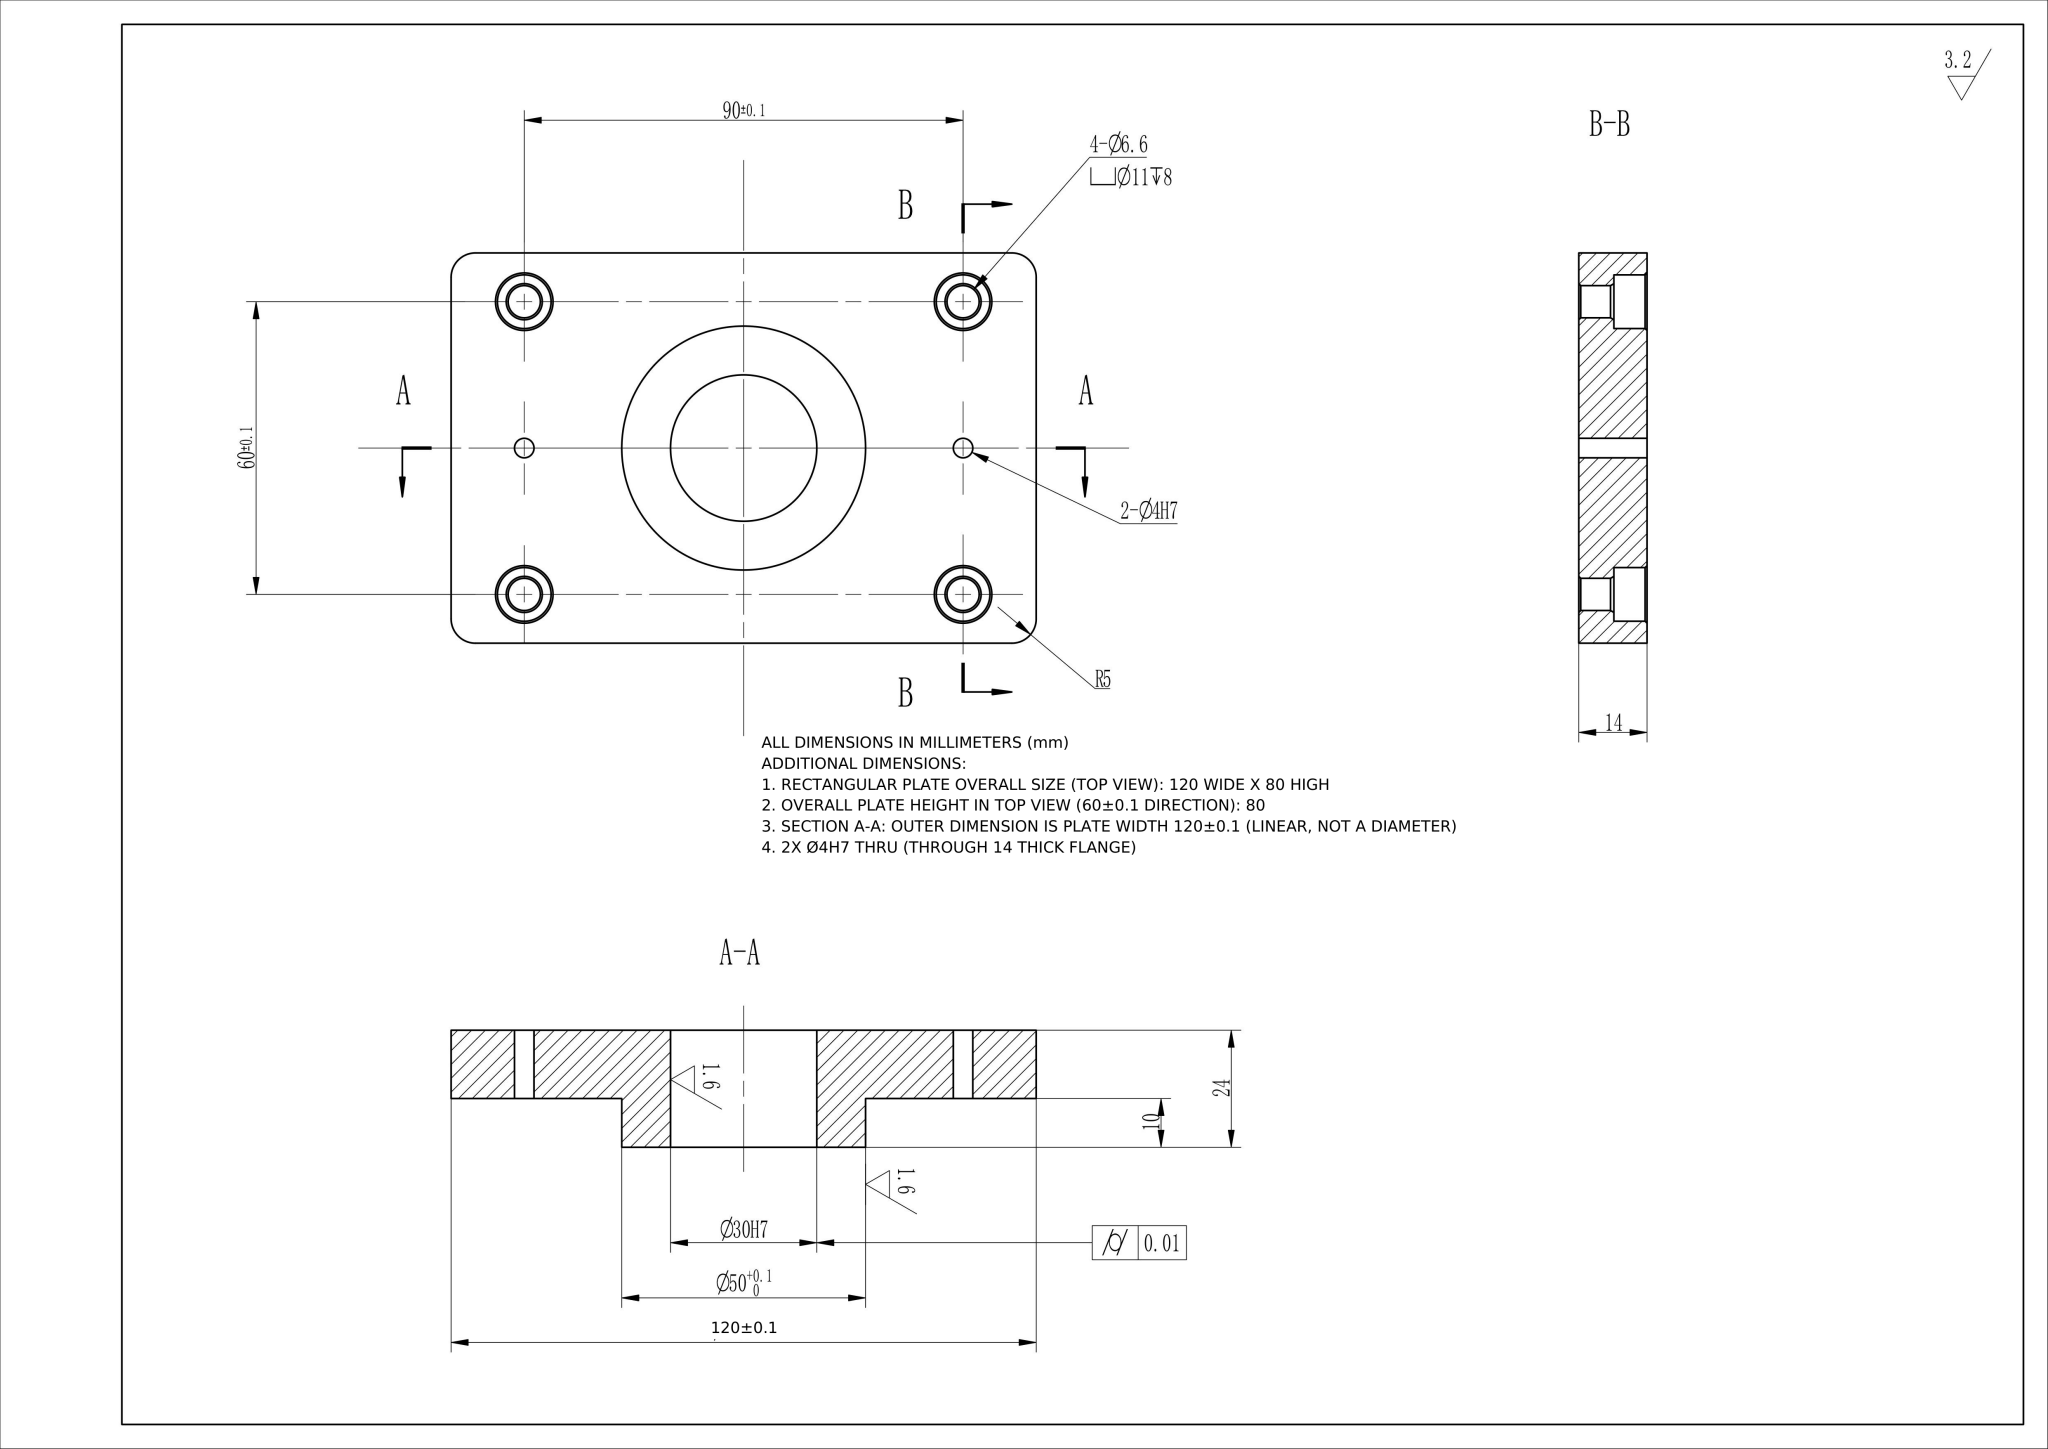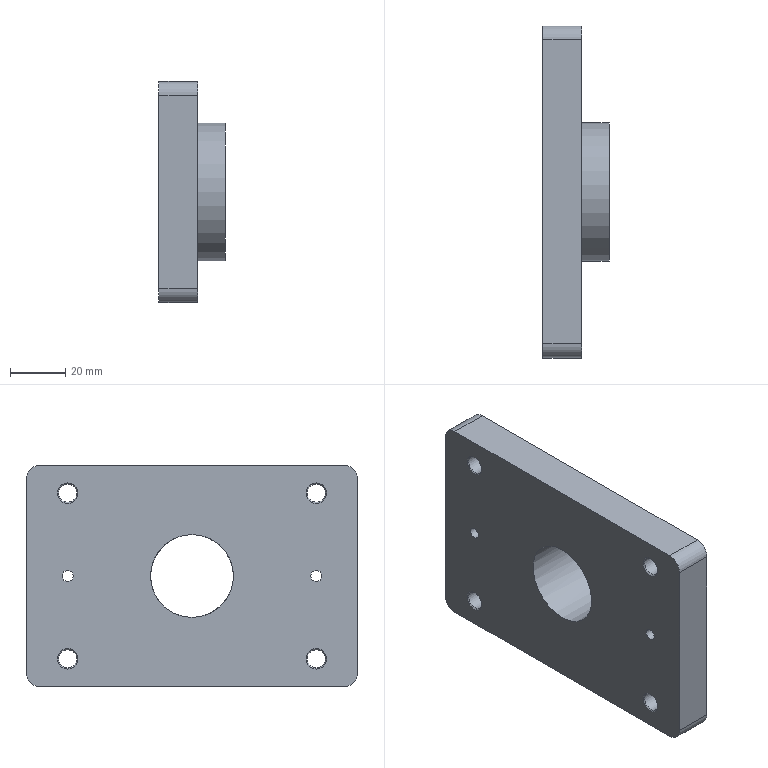Part | NX | mm | 1 solid | 39 faces | box 24 x 120 x 80 mm | volume 132818 mm3 | cylinder 16 | cone 12 | plane 11 | commonest cylinder face diameters 6.6 x4 11 x4 10 x4 4 x2 50 x1 30 x1
STEP:
#1=CARTESIAN_POINT('',(0.,0.,0.));
#2=DIRECTION('',(0.,0.,1.));
#3=DIRECTION('',(1.,0.,0.));
#4=AXIS2_PLACEMENT_3D('',#1,#2,#3);
#5=(LENGTH_UNIT()NAMED_UNIT(*)SI_UNIT(.MILLI.,.METRE.));
#6=UNCERTAINTY_MEASURE_WITH_UNIT(LENGTH_MEASURE(0.00002),#5,'','');
#7=(NAMED_UNIT(*)PLANE_ANGLE_UNIT()SI_UNIT($,.RADIAN.));
#8=PLANE_ANGLE_MEASURE_WITH_UNIT(PLANE_ANGLE_MEASURE(0.01745),#7);
#9=DIMENSIONAL_EXPONENTS(0.,0.,0.,0.,0.,0.,0.);
#10=(CONVERSION_BASED_UNIT('',#8)NAMED_UNIT(#9)PLANE_ANGLE_UNIT());
#11=(NAMED_UNIT(*)SI_UNIT($,.STERADIAN.)SOLID_ANGLE_UNIT());
#12=(GEOMETRIC_REPRESENTATION_CONTEXT(3)GLOBAL_UNCERTAINTY_ASSIGNED_CONTEXT((#6))GLOBAL_UNIT_ASSIGNED_CONTEXT((#5,#10,#11))REPRESENTATION_CONTEXT('',''));
#13=SHAPE_REPRESENTATION('',(#4),#12);
#14=CARTESIAN_POINT('',(0.,-60.,35.));
#15=VERTEX_POINT('',#14);
#16=CARTESIAN_POINT('',(0.,-60.,-35.));
#17=VERTEX_POINT('',#16);
#18=CARTESIAN_POINT('',(0.,-60.,40.));
#19=DIRECTION('',(0.,0.,-1.));
#20=VECTOR('',#19,1.);
#21=LINE('',#18,#20);
#22=EDGE_CURVE('',#15,#17,#21,.T.);
#23=ORIENTED_EDGE('',*,*,#22,.T.);
#24=CARTESIAN_POINT('',(14.,-60.,-35.));
#25=VERTEX_POINT('',#24);
#26=CARTESIAN_POINT('',(14.,-60.,-35.));
#27=DIRECTION('',(1.,0.,0.));
#28=VECTOR('',#27,1.);
#29=LINE('',#26,#28);
#30=EDGE_CURVE('',#17,#25,#29,.T.);
#31=ORIENTED_EDGE('',*,*,#30,.T.);
#32=CARTESIAN_POINT('',(14.,-60.,35.));
#33=VERTEX_POINT('',#32);
#34=CARTESIAN_POINT('',(14.,-60.,40.));
#35=DIRECTION('',(0.,0.,-1.));
#36=VECTOR('',#35,1.);
#37=LINE('',#34,#36);
#38=EDGE_CURVE('',#33,#25,#37,.T.);
#39=ORIENTED_EDGE('',*,*,#38,.F.);
#40=CARTESIAN_POINT('',(14.,-60.,35.));
#41=DIRECTION('',(-1.,0.,0.));
#42=VECTOR('',#41,1.);
#43=LINE('',#40,#42);
#44=EDGE_CURVE('',#33,#15,#43,.T.);
#45=ORIENTED_EDGE('',*,*,#44,.T.);
#46=EDGE_LOOP('',(#23,#31,#39,#45));
#47=FACE_OUTER_BOUND('',#46,.T.);
#48=CARTESIAN_POINT('',(14.,-60.,40.));
#49=DIRECTION('',(0.,1.,0.));
#50=DIRECTION('',(0.,0.,1.));
#51=AXIS2_PLACEMENT_3D('',#48,#49,#50);
#52=PLANE('',#51);
#53=ADVANCED_FACE('',(#47),#52,.F.);
#54=CARTESIAN_POINT('',(0.,-55.,-40.));
#55=VERTEX_POINT('',#54);
#56=CARTESIAN_POINT('',(0.,55.,-40.));
#57=VERTEX_POINT('',#56);
#58=CARTESIAN_POINT('',(0.,-60.,-40.));
#59=DIRECTION('',(0.,1.,0.));
#60=VECTOR('',#59,1.);
#61=LINE('',#58,#60);
#62=EDGE_CURVE('',#55,#57,#61,.T.);
#63=ORIENTED_EDGE('',*,*,#62,.T.);
#64=CARTESIAN_POINT('',(14.,55.,-40.));
#65=VERTEX_POINT('',#64);
#66=CARTESIAN_POINT('',(14.,55.,-40.));
#67=DIRECTION('',(1.,0.,0.));
#68=VECTOR('',#67,1.);
#69=LINE('',#66,#68);
#70=EDGE_CURVE('',#57,#65,#69,.T.);
#71=ORIENTED_EDGE('',*,*,#70,.T.);
#72=CARTESIAN_POINT('',(14.,-55.,-40.));
#73=VERTEX_POINT('',#72);
#74=CARTESIAN_POINT('',(14.,-60.,-40.));
#75=DIRECTION('',(0.,1.,0.));
#76=VECTOR('',#75,1.);
#77=LINE('',#74,#76);
#78=EDGE_CURVE('',#73,#65,#77,.T.);
#79=ORIENTED_EDGE('',*,*,#78,.F.);
#80=CARTESIAN_POINT('',(14.,-55.,-40.));
#81=DIRECTION('',(-1.,0.,0.));
#82=VECTOR('',#81,1.);
#83=LINE('',#80,#82);
#84=EDGE_CURVE('',#73,#55,#83,.T.);
#85=ORIENTED_EDGE('',*,*,#84,.T.);
#86=EDGE_LOOP('',(#63,#71,#79,#85));
#87=FACE_OUTER_BOUND('',#86,.T.);
#88=CARTESIAN_POINT('',(14.,-60.,-40.));
#89=DIRECTION('',(0.,0.,1.));
#90=DIRECTION('',(1.,0.,0.));
#91=AXIS2_PLACEMENT_3D('',#88,#89,#90);
#92=PLANE('',#91);
#93=ADVANCED_FACE('',(#87),#92,.F.);
#94=CARTESIAN_POINT('',(14.,60.,-35.));
#95=VERTEX_POINT('',#94);
#96=CARTESIAN_POINT('',(14.,60.,35.));
#97=VERTEX_POINT('',#96);
#98=CARTESIAN_POINT('',(14.,60.,-40.));
#99=DIRECTION('',(0.,0.,1.));
#100=VECTOR('',#99,1.);
#101=LINE('',#98,#100);
#102=EDGE_CURVE('',#95,#97,#101,.T.);
#103=ORIENTED_EDGE('',*,*,#102,.F.);
#104=CARTESIAN_POINT('',(0.,60.,-35.));
#105=VERTEX_POINT('',#104);
#106=CARTESIAN_POINT('',(14.,60.,-35.));
#107=DIRECTION('',(-1.,0.,0.));
#108=VECTOR('',#107,1.);
#109=LINE('',#106,#108);
#110=EDGE_CURVE('',#95,#105,#109,.T.);
#111=ORIENTED_EDGE('',*,*,#110,.T.);
#112=CARTESIAN_POINT('',(0.,60.,35.));
#113=VERTEX_POINT('',#112);
#114=CARTESIAN_POINT('',(0.,60.,-40.));
#115=DIRECTION('',(0.,0.,1.));
#116=VECTOR('',#115,1.);
#117=LINE('',#114,#116);
#118=EDGE_CURVE('',#105,#113,#117,.T.);
#119=ORIENTED_EDGE('',*,*,#118,.T.);
#120=CARTESIAN_POINT('',(14.,60.,35.));
#121=DIRECTION('',(1.,0.,0.));
#122=VECTOR('',#121,1.);
#123=LINE('',#120,#122);
#124=EDGE_CURVE('',#113,#97,#123,.T.);
#125=ORIENTED_EDGE('',*,*,#124,.T.);
#126=EDGE_LOOP('',(#103,#111,#119,#125));
#127=FACE_OUTER_BOUND('',#126,.T.);
#128=CARTESIAN_POINT('',(14.,60.,-40.));
#129=DIRECTION('',(0.,-1.,0.));
#130=DIRECTION('',(0.,0.,-1.));
#131=AXIS2_PLACEMENT_3D('',#128,#129,#130);
#132=PLANE('',#131);
#133=ADVANCED_FACE('',(#127),#132,.F.);
#134=CARTESIAN_POINT('',(14.,55.,40.));
#135=VERTEX_POINT('',#134);
#136=CARTESIAN_POINT('',(14.,-55.,40.));
#137=VERTEX_POINT('',#136);
#138=CARTESIAN_POINT('',(14.,60.,40.));
#139=DIRECTION('',(0.,-1.,0.));
#140=VECTOR('',#139,1.);
#141=LINE('',#138,#140);
#142=EDGE_CURVE('',#135,#137,#141,.T.);
#143=ORIENTED_EDGE('',*,*,#142,.F.);
#144=CARTESIAN_POINT('',(0.,55.,40.));
#145=VERTEX_POINT('',#144);
#146=CARTESIAN_POINT('',(14.,55.,40.));
#147=DIRECTION('',(-1.,0.,0.));
#148=VECTOR('',#147,1.);
#149=LINE('',#146,#148);
#150=EDGE_CURVE('',#135,#145,#149,.T.);
#151=ORIENTED_EDGE('',*,*,#150,.T.);
#152=CARTESIAN_POINT('',(0.,-55.,40.));
#153=VERTEX_POINT('',#152);
#154=CARTESIAN_POINT('',(0.,60.,40.));
#155=DIRECTION('',(0.,-1.,0.));
#156=VECTOR('',#155,1.);
#157=LINE('',#154,#156);
#158=EDGE_CURVE('',#145,#153,#157,.T.);
#159=ORIENTED_EDGE('',*,*,#158,.T.);
#160=CARTESIAN_POINT('',(14.,-55.,40.));
#161=DIRECTION('',(1.,0.,0.));
#162=VECTOR('',#161,1.);
#163=LINE('',#160,#162);
#164=EDGE_CURVE('',#153,#137,#163,.T.);
#165=ORIENTED_EDGE('',*,*,#164,.T.);
#166=EDGE_LOOP('',(#143,#151,#159,#165));
#167=FACE_OUTER_BOUND('',#166,.T.);
#168=CARTESIAN_POINT('',(14.,60.,40.));
#169=DIRECTION('',(0.,0.,-1.));
#170=DIRECTION('',(-1.,0.,0.));
#171=AXIS2_PLACEMENT_3D('',#168,#169,#170);
#172=PLANE('',#171);
#173=ADVANCED_FACE('',(#167),#172,.F.);
#174=CARTESIAN_POINT('',(14.,45.,2.));
#175=VERTEX_POINT('',#174);
#176=CARTESIAN_POINT('',(14.,45.,0.));
#177=DIRECTION('',(-1.,0.,0.));
#178=DIRECTION('',(0.,0.,1.));
#179=AXIS2_PLACEMENT_3D('',#176,#177,#178);
#180=CIRCLE('',#179,2.);
#181=EDGE_CURVE('',#175,#175,#180,.T.);
#182=ORIENTED_EDGE('',*,*,#181,.T.);
#183=EDGE_LOOP('',(#182));
#184=FACE_BOUND('',#183,.T.);
#185=CARTESIAN_POINT('',(14.,-45.,2.));
#186=VERTEX_POINT('',#185);
#187=CARTESIAN_POINT('',(14.,-45.,0.));
#188=DIRECTION('',(-1.,0.,0.));
#189=DIRECTION('',(0.,0.,1.));
#190=AXIS2_PLACEMENT_3D('',#187,#188,#189);
#191=CIRCLE('',#190,2.);
#192=EDGE_CURVE('',#186,#186,#191,.T.);
#193=ORIENTED_EDGE('',*,*,#192,.T.);
#194=EDGE_LOOP('',(#193));
#195=FACE_BOUND('',#194,.T.);
#196=CARTESIAN_POINT('',(14.,25.,-0.));
#197=VERTEX_POINT('',#196);
#198=CARTESIAN_POINT('',(14.,0.,0.));
#199=DIRECTION('',(1.,0.,0.));
#200=DIRECTION('',(0.,1.,-0.));
#201=AXIS2_PLACEMENT_3D('',#198,#199,#200);
#202=CIRCLE('',#201,25.);
#203=EDGE_CURVE('',#197,#197,#202,.T.);
#204=ORIENTED_EDGE('',*,*,#203,.F.);
#205=EDGE_LOOP('',(#204));
#206=FACE_BOUND('',#205,.T.);
#207=CARTESIAN_POINT('',(14.,45.,-35.9));
#208=VERTEX_POINT('',#207);
#209=CARTESIAN_POINT('',(14.,45.,-30.));
#210=DIRECTION('',(-1.,0.,0.));
#211=DIRECTION('',(0.,0.,-1.));
#212=AXIS2_PLACEMENT_3D('',#209,#210,#211);
#213=CIRCLE('',#212,5.9);
#214=EDGE_CURVE('',#208,#208,#213,.T.);
#215=ORIENTED_EDGE('',*,*,#214,.T.);
#216=EDGE_LOOP('',(#215));
#217=FACE_BOUND('',#216,.T.);
#218=CARTESIAN_POINT('',(14.,-45.,-35.9));
#219=VERTEX_POINT('',#218);
#220=CARTESIAN_POINT('',(14.,-45.,-30.));
#221=DIRECTION('',(-1.,0.,0.));
#222=DIRECTION('',(0.,0.,-1.));
#223=AXIS2_PLACEMENT_3D('',#220,#221,#222);
#224=CIRCLE('',#223,5.9);
#225=EDGE_CURVE('',#219,#219,#224,.T.);
#226=ORIENTED_EDGE('',*,*,#225,.T.);
#227=EDGE_LOOP('',(#226));
#228=FACE_BOUND('',#227,.T.);
#229=CARTESIAN_POINT('',(14.,45.,24.1));
#230=VERTEX_POINT('',#229);
#231=CARTESIAN_POINT('',(14.,45.,30.));
#232=DIRECTION('',(-1.,0.,0.));
#233=DIRECTION('',(0.,0.,-1.));
#234=AXIS2_PLACEMENT_3D('',#231,#232,#233);
#235=CIRCLE('',#234,5.9);
#236=EDGE_CURVE('',#230,#230,#235,.T.);
#237=ORIENTED_EDGE('',*,*,#236,.T.);
#238=EDGE_LOOP('',(#237));
#239=FACE_BOUND('',#238,.T.);
#240=CARTESIAN_POINT('',(14.,-45.,24.1));
#241=VERTEX_POINT('',#240);
#242=CARTESIAN_POINT('',(14.,-45.,30.));
#243=DIRECTION('',(-1.,0.,0.));
#244=DIRECTION('',(0.,0.,-1.));
#245=AXIS2_PLACEMENT_3D('',#242,#243,#244);
#246=CIRCLE('',#245,5.9);
#247=EDGE_CURVE('',#241,#241,#246,.T.);
#248=ORIENTED_EDGE('',*,*,#247,.T.);
#249=EDGE_LOOP('',(#248));
#250=FACE_BOUND('',#249,.T.);
#251=ORIENTED_EDGE('',*,*,#78,.T.);
#252=CARTESIAN_POINT('',(14.,55.,-35.));
#253=DIRECTION('',(1.,0.,0.));
#254=DIRECTION('',(0.,0.,-1.));
#255=AXIS2_PLACEMENT_3D('',#252,#253,#254);
#256=CIRCLE('',#255,5.);
#257=EDGE_CURVE('',#65,#95,#256,.T.);
#258=ORIENTED_EDGE('',*,*,#257,.T.);
#259=ORIENTED_EDGE('',*,*,#102,.T.);
#260=CARTESIAN_POINT('',(14.,55.,35.));
#261=DIRECTION('',(1.,0.,0.));
#262=DIRECTION('',(0.,0.,-1.));
#263=AXIS2_PLACEMENT_3D('',#260,#261,#262);
#264=CIRCLE('',#263,5.);
#265=EDGE_CURVE('',#97,#135,#264,.T.);
#266=ORIENTED_EDGE('',*,*,#265,.T.);
#267=ORIENTED_EDGE('',*,*,#142,.T.);
#268=CARTESIAN_POINT('',(14.,-55.,35.));
#269=DIRECTION('',(1.,0.,0.));
#270=DIRECTION('',(0.,0.,-1.));
#271=AXIS2_PLACEMENT_3D('',#268,#269,#270);
#272=CIRCLE('',#271,5.);
#273=EDGE_CURVE('',#137,#33,#272,.T.);
#274=ORIENTED_EDGE('',*,*,#273,.T.);
#275=ORIENTED_EDGE('',*,*,#38,.T.);
#276=CARTESIAN_POINT('',(14.,-55.,-35.));
#277=DIRECTION('',(1.,0.,0.));
#278=DIRECTION('',(0.,0.,-1.));
#279=AXIS2_PLACEMENT_3D('',#276,#277,#278);
#280=CIRCLE('',#279,5.);
#281=EDGE_CURVE('',#25,#73,#280,.T.);
#282=ORIENTED_EDGE('',*,*,#281,.T.);
#283=EDGE_LOOP('',(#251,#258,#259,#266,#267,#274,#275,#282));
#284=FACE_BOUND('',#283,.T.);
#285=CARTESIAN_POINT('',(14.,0.,0.));
#286=DIRECTION('',(1.,0.,0.));
#287=DIRECTION('',(0.,0.,-1.));
#288=AXIS2_PLACEMENT_3D('',#285,#286,#287);
#289=PLANE('',#288);
#290=ADVANCED_FACE('',(#184,#195,#206,#217,#228,#239,#250,#284),#289,.T.);
#291=CARTESIAN_POINT('',(0.,45.,-2.));
#292=VERTEX_POINT('',#291);
#293=CARTESIAN_POINT('',(0.,45.,0.));
#294=DIRECTION('',(1.,0.,0.));
#295=DIRECTION('',(0.,0.,-1.));
#296=AXIS2_PLACEMENT_3D('',#293,#294,#295);
#297=CIRCLE('',#296,2.);
#298=EDGE_CURVE('',#292,#292,#297,.T.);
#299=ORIENTED_EDGE('',*,*,#298,.T.);
#300=EDGE_LOOP('',(#299));
#301=FACE_BOUND('',#300,.T.);
#302=CARTESIAN_POINT('',(0.,-45.,-2.));
#303=VERTEX_POINT('',#302);
#304=CARTESIAN_POINT('',(0.,-45.,0.));
#305=DIRECTION('',(1.,0.,0.));
#306=DIRECTION('',(0.,0.,-1.));
#307=AXIS2_PLACEMENT_3D('',#304,#305,#306);
#308=CIRCLE('',#307,2.);
#309=EDGE_CURVE('',#303,#303,#308,.T.);
#310=ORIENTED_EDGE('',*,*,#309,.T.);
#311=EDGE_LOOP('',(#310));
#312=FACE_BOUND('',#311,.T.);
#313=CARTESIAN_POINT('',(0.,0.,-15.));
#314=VERTEX_POINT('',#313);
#315=CARTESIAN_POINT('',(0.,0.,0.));
#316=DIRECTION('',(1.,0.,0.));
#317=DIRECTION('',(0.,0.,-1.));
#318=AXIS2_PLACEMENT_3D('',#315,#316,#317);
#319=CIRCLE('',#318,15.);
#320=EDGE_CURVE('',#314,#314,#319,.T.);
#321=ORIENTED_EDGE('',*,*,#320,.T.);
#322=EDGE_LOOP('',(#321));
#323=FACE_BOUND('',#322,.T.);
#324=CARTESIAN_POINT('',(0.,45.,-33.7));
#325=VERTEX_POINT('',#324);
#326=CARTESIAN_POINT('',(0.,45.,-30.));
#327=DIRECTION('',(1.,0.,0.));
#328=DIRECTION('',(0.,0.,-1.));
#329=AXIS2_PLACEMENT_3D('',#326,#327,#328);
#330=CIRCLE('',#329,3.7);
#331=EDGE_CURVE('',#325,#325,#330,.T.);
#332=ORIENTED_EDGE('',*,*,#331,.T.);
#333=EDGE_LOOP('',(#332));
#334=FACE_BOUND('',#333,.T.);
#335=CARTESIAN_POINT('',(0.,-45.,-33.7));
#336=VERTEX_POINT('',#335);
#337=CARTESIAN_POINT('',(0.,-45.,-30.));
#338=DIRECTION('',(1.,0.,0.));
#339=DIRECTION('',(0.,0.,-1.));
#340=AXIS2_PLACEMENT_3D('',#337,#338,#339);
#341=CIRCLE('',#340,3.7);
#342=EDGE_CURVE('',#336,#336,#341,.T.);
#343=ORIENTED_EDGE('',*,*,#342,.T.);
#344=EDGE_LOOP('',(#343));
#345=FACE_BOUND('',#344,.T.);
#346=CARTESIAN_POINT('',(0.,45.,26.3));
#347=VERTEX_POINT('',#346);
#348=CARTESIAN_POINT('',(0.,45.,30.));
#349=DIRECTION('',(1.,0.,0.));
#350=DIRECTION('',(0.,0.,-1.));
#351=AXIS2_PLACEMENT_3D('',#348,#349,#350);
#352=CIRCLE('',#351,3.7);
#353=EDGE_CURVE('',#347,#347,#352,.T.);
#354=ORIENTED_EDGE('',*,*,#353,.T.);
#355=EDGE_LOOP('',(#354));
#356=FACE_BOUND('',#355,.T.);
#357=CARTESIAN_POINT('',(0.,-45.,26.3));
#358=VERTEX_POINT('',#357);
#359=CARTESIAN_POINT('',(0.,-45.,30.));
#360=DIRECTION('',(1.,0.,0.));
#361=DIRECTION('',(0.,0.,-1.));
#362=AXIS2_PLACEMENT_3D('',#359,#360,#361);
#363=CIRCLE('',#362,3.7);
#364=EDGE_CURVE('',#358,#358,#363,.T.);
#365=ORIENTED_EDGE('',*,*,#364,.T.);
#366=EDGE_LOOP('',(#365));
#367=FACE_BOUND('',#366,.T.);
#368=ORIENTED_EDGE('',*,*,#118,.F.);
#369=CARTESIAN_POINT('',(0.,55.,-35.));
#370=DIRECTION('',(-1.,0.,0.));
#371=DIRECTION('',(0.,0.,-1.));
#372=AXIS2_PLACEMENT_3D('',#369,#370,#371);
#373=CIRCLE('',#372,5.);
#374=EDGE_CURVE('',#105,#57,#373,.T.);
#375=ORIENTED_EDGE('',*,*,#374,.T.);
#376=ORIENTED_EDGE('',*,*,#62,.F.);
#377=CARTESIAN_POINT('',(0.,-55.,-35.));
#378=DIRECTION('',(-1.,0.,0.));
#379=DIRECTION('',(0.,0.,-1.));
#380=AXIS2_PLACEMENT_3D('',#377,#378,#379);
#381=CIRCLE('',#380,5.);
#382=EDGE_CURVE('',#55,#17,#381,.T.);
#383=ORIENTED_EDGE('',*,*,#382,.T.);
#384=ORIENTED_EDGE('',*,*,#22,.F.);
#385=CARTESIAN_POINT('',(0.,-55.,35.));
#386=DIRECTION('',(-1.,0.,0.));
#387=DIRECTION('',(0.,0.,-1.));
#388=AXIS2_PLACEMENT_3D('',#385,#386,#387);
#389=CIRCLE('',#388,5.);
#390=EDGE_CURVE('',#15,#153,#389,.T.);
#391=ORIENTED_EDGE('',*,*,#390,.T.);
#392=ORIENTED_EDGE('',*,*,#158,.F.);
#393=CARTESIAN_POINT('',(0.,55.,35.));
#394=DIRECTION('',(-1.,0.,0.));
#395=DIRECTION('',(0.,0.,-1.));
#396=AXIS2_PLACEMENT_3D('',#393,#394,#395);
#397=CIRCLE('',#396,5.);
#398=EDGE_CURVE('',#145,#113,#397,.T.);
#399=ORIENTED_EDGE('',*,*,#398,.T.);
#400=EDGE_LOOP('',(#368,#375,#376,#383,#384,#391,#392,#399));
#401=FACE_BOUND('',#400,.T.);
#402=CARTESIAN_POINT('',(0.,0.,0.));
#403=DIRECTION('',(1.,0.,0.));
#404=DIRECTION('',(0.,0.,-1.));
#405=AXIS2_PLACEMENT_3D('',#402,#403,#404);
#406=PLANE('',#405);
#407=ADVANCED_FACE('',(#301,#312,#323,#334,#345,#356,#367,#401),#406,.F.);
#408=CARTESIAN_POINT('',(0.4,-45.,26.7));
#409=VERTEX_POINT('',#408);
#410=CARTESIAN_POINT('',(0.4,-45.,30.));
#411=DIRECTION('',(-1.,0.,0.));
#412=DIRECTION('',(0.,0.,-1.));
#413=AXIS2_PLACEMENT_3D('',#410,#411,#412);
#414=CIRCLE('',#413,3.3);
#415=EDGE_CURVE('',#409,#409,#414,.T.);
#416=ORIENTED_EDGE('',*,*,#415,.T.);
#417=EDGE_LOOP('',(#416));
#418=FACE_BOUND('',#417,.T.);
#419=CARTESIAN_POINT('',(6.507,-45.,33.3));
#420=VERTEX_POINT('',#419);
#421=CARTESIAN_POINT('',(6.507,-45.,30.));
#422=DIRECTION('',(1.,0.,0.));
#423=DIRECTION('',(0.,0.,1.));
#424=AXIS2_PLACEMENT_3D('',#421,#422,#423);
#425=CIRCLE('',#424,3.3);
#426=EDGE_CURVE('',#420,#420,#425,.T.);
#427=ORIENTED_EDGE('',*,*,#426,.T.);
#428=EDGE_LOOP('',(#427));
#429=FACE_BOUND('',#428,.T.);
#430=CARTESIAN_POINT('',(-36.,-45.,30.));
#431=DIRECTION('',(-1.,0.,0.));
#432=DIRECTION('',(0.,0.,1.));
#433=AXIS2_PLACEMENT_3D('',#430,#431,#432);
#434=CYLINDRICAL_SURFACE('',#433,3.3);
#435=ADVANCED_FACE('',(#418,#429),#434,.F.);
#436=CARTESIAN_POINT('',(7.2,-45.,33.7));
#437=VERTEX_POINT('',#436);
#438=CARTESIAN_POINT('',(7.2,-45.,30.));
#439=DIRECTION('',(-1.,0.,0.));
#440=DIRECTION('',(0.,0.,1.));
#441=AXIS2_PLACEMENT_3D('',#438,#439,#440);
#442=CIRCLE('',#441,3.7);
#443=EDGE_CURVE('',#437,#437,#442,.T.);
#444=ORIENTED_EDGE('',*,*,#443,.T.);
#445=EDGE_LOOP('',(#444));
#446=FACE_BOUND('',#445,.T.);
#447=CARTESIAN_POINT('',(7.2,-45.,35.5));
#448=VERTEX_POINT('',#447);
#449=CARTESIAN_POINT('',(7.2,-45.,30.));
#450=DIRECTION('',(1.,0.,0.));
#451=DIRECTION('',(0.,0.,1.));
#452=AXIS2_PLACEMENT_3D('',#449,#450,#451);
#453=CIRCLE('',#452,5.5);
#454=EDGE_CURVE('',#448,#448,#453,.T.);
#455=ORIENTED_EDGE('',*,*,#454,.T.);
#456=EDGE_LOOP('',(#455));
#457=FACE_BOUND('',#456,.T.);
#458=CARTESIAN_POINT('',(7.2,-45.,30.));
#459=DIRECTION('',(-1.,0.,0.));
#460=DIRECTION('',(0.,0.,1.));
#461=AXIS2_PLACEMENT_3D('',#458,#459,#460);
#462=PLANE('',#461);
#463=ADVANCED_FACE('',(#446,#457),#462,.F.);
#464=CARTESIAN_POINT('',(13.6,-45.,24.5));
#465=VERTEX_POINT('',#464);
#466=CARTESIAN_POINT('',(13.6,-45.,30.));
#467=DIRECTION('',(1.,0.,0.));
#468=DIRECTION('',(0.,0.,-1.));
#469=AXIS2_PLACEMENT_3D('',#466,#467,#468);
#470=CIRCLE('',#469,5.5);
#471=EDGE_CURVE('',#465,#465,#470,.T.);
#472=ORIENTED_EDGE('',*,*,#471,.T.);
#473=EDGE_LOOP('',(#472));
#474=FACE_BOUND('',#473,.T.);
#475=ORIENTED_EDGE('',*,*,#454,.F.);
#476=EDGE_LOOP('',(#475));
#477=FACE_BOUND('',#476,.T.);
#478=CARTESIAN_POINT('',(14.,-45.,30.));
#479=DIRECTION('',(-1.,0.,0.));
#480=DIRECTION('',(0.,0.,1.));
#481=AXIS2_PLACEMENT_3D('',#478,#479,#480);
#482=CYLINDRICAL_SURFACE('',#481,5.5);
#483=ADVANCED_FACE('',(#474,#477),#482,.F.);
#484=ORIENTED_EDGE('',*,*,#443,.F.);
#485=EDGE_LOOP('',(#484));
#486=FACE_BOUND('',#485,.T.);
#487=ORIENTED_EDGE('',*,*,#426,.F.);
#488=EDGE_LOOP('',(#487));
#489=FACE_BOUND('',#488,.T.);
#490=CARTESIAN_POINT('',(6.507,-45.,30.));
#491=DIRECTION('',(1.,0.,0.));
#492=DIRECTION('',(0.,0.,-1.));
#493=AXIS2_PLACEMENT_3D('',#490,#491,#492);
#494=CONICAL_SURFACE('',#493,3.3,30.);
#495=ADVANCED_FACE('',(#486,#489),#494,.F.);
#496=ORIENTED_EDGE('',*,*,#471,.F.);
#497=EDGE_LOOP('',(#496));
#498=FACE_BOUND('',#497,.T.);
#499=ORIENTED_EDGE('',*,*,#247,.F.);
#500=EDGE_LOOP('',(#499));
#501=FACE_BOUND('',#500,.T.);
#502=CARTESIAN_POINT('',(14.,-45.,30.));
#503=DIRECTION('',(1.,0.,0.));
#504=DIRECTION('',(-0.,0.,-1.));
#505=AXIS2_PLACEMENT_3D('',#502,#503,#504);
#506=CONICAL_SURFACE('',#505,5.9,45.);
#507=ADVANCED_FACE('',(#498,#501),#506,.F.);
#508=ORIENTED_EDGE('',*,*,#415,.F.);
#509=EDGE_LOOP('',(#508));
#510=FACE_BOUND('',#509,.T.);
#511=ORIENTED_EDGE('',*,*,#364,.F.);
#512=EDGE_LOOP('',(#511));
#513=FACE_BOUND('',#512,.T.);
#514=CARTESIAN_POINT('',(0.,-45.,30.));
#515=DIRECTION('',(-1.,0.,0.));
#516=DIRECTION('',(0.,0.,1.));
#517=AXIS2_PLACEMENT_3D('',#514,#515,#516);
#518=CONICAL_SURFACE('',#517,3.7,45.);
#519=ADVANCED_FACE('',(#510,#513),#518,.F.);
#520=CARTESIAN_POINT('',(0.4,45.,26.7));
#521=VERTEX_POINT('',#520);
#522=CARTESIAN_POINT('',(0.4,45.,30.));
#523=DIRECTION('',(-1.,0.,0.));
#524=DIRECTION('',(0.,0.,-1.));
#525=AXIS2_PLACEMENT_3D('',#522,#523,#524);
#526=CIRCLE('',#525,3.3);
#527=EDGE_CURVE('',#521,#521,#526,.T.);
#528=ORIENTED_EDGE('',*,*,#527,.T.);
#529=EDGE_LOOP('',(#528));
#530=FACE_BOUND('',#529,.T.);
#531=CARTESIAN_POINT('',(6.507,45.,33.3));
#532=VERTEX_POINT('',#531);
#533=CARTESIAN_POINT('',(6.507,45.,30.));
#534=DIRECTION('',(1.,0.,0.));
#535=DIRECTION('',(0.,0.,1.));
#536=AXIS2_PLACEMENT_3D('',#533,#534,#535);
#537=CIRCLE('',#536,3.3);
#538=EDGE_CURVE('',#532,#532,#537,.T.);
#539=ORIENTED_EDGE('',*,*,#538,.T.);
#540=EDGE_LOOP('',(#539));
#541=FACE_BOUND('',#540,.T.);
#542=CARTESIAN_POINT('',(-36.,45.,30.));
#543=DIRECTION('',(-1.,0.,0.));
#544=DIRECTION('',(0.,0.,1.));
#545=AXIS2_PLACEMENT_3D('',#542,#543,#544);
#546=CYLINDRICAL_SURFACE('',#545,3.3);
#547=ADVANCED_FACE('',(#530,#541),#546,.F.);
#548=CARTESIAN_POINT('',(7.2,45.,33.7));
#549=VERTEX_POINT('',#548);
#550=CARTESIAN_POINT('',(7.2,45.,30.));
#551=DIRECTION('',(-1.,0.,0.));
#552=DIRECTION('',(0.,0.,1.));
#553=AXIS2_PLACEMENT_3D('',#550,#551,#552);
#554=CIRCLE('',#553,3.7);
#555=EDGE_CURVE('',#549,#549,#554,.T.);
#556=ORIENTED_EDGE('',*,*,#555,.T.);
#557=EDGE_LOOP('',(#556));
#558=FACE_BOUND('',#557,.T.);
#559=CARTESIAN_POINT('',(7.2,45.,35.5));
#560=VERTEX_POINT('',#559);
#561=CARTESIAN_POINT('',(7.2,45.,30.));
#562=DIRECTION('',(1.,0.,0.));
#563=DIRECTION('',(0.,0.,1.));
#564=AXIS2_PLACEMENT_3D('',#561,#562,#563);
#565=CIRCLE('',#564,5.5);
#566=EDGE_CURVE('',#560,#560,#565,.T.);
#567=ORIENTED_EDGE('',*,*,#566,.T.);
#568=EDGE_LOOP('',(#567));
#569=FACE_BOUND('',#568,.T.);
#570=CARTESIAN_POINT('',(7.2,45.,30.));
#571=DIRECTION('',(-1.,0.,0.));
#572=DIRECTION('',(0.,0.,1.));
#573=AXIS2_PLACEMENT_3D('',#570,#571,#572);
#574=PLANE('',#573);
#575=ADVANCED_FACE('',(#558,#569),#574,.F.);
#576=CARTESIAN_POINT('',(13.6,45.,24.5));
#577=VERTEX_POINT('',#576);
#578=CARTESIAN_POINT('',(13.6,45.,30.));
#579=DIRECTION('',(1.,0.,0.));
#580=DIRECTION('',(0.,0.,-1.));
#581=AXIS2_PLACEMENT_3D('',#578,#579,#580);
#582=CIRCLE('',#581,5.5);
#583=EDGE_CURVE('',#577,#577,#582,.T.);
#584=ORIENTED_EDGE('',*,*,#583,.T.);
#585=EDGE_LOOP('',(#584));
#586=FACE_BOUND('',#585,.T.);
#587=ORIENTED_EDGE('',*,*,#566,.F.);
#588=EDGE_LOOP('',(#587));
#589=FACE_BOUND('',#588,.T.);
#590=CARTESIAN_POINT('',(14.,45.,30.));
#591=DIRECTION('',(-1.,0.,0.));
#592=DIRECTION('',(0.,0.,1.));
#593=AXIS2_PLACEMENT_3D('',#590,#591,#592);
#594=CYLINDRICAL_SURFACE('',#593,5.5);
#595=ADVANCED_FACE('',(#586,#589),#594,.F.);
#596=ORIENTED_EDGE('',*,*,#555,.F.);
#597=EDGE_LOOP('',(#596));
#598=FACE_BOUND('',#597,.T.);
#599=ORIENTED_EDGE('',*,*,#538,.F.);
#600=EDGE_LOOP('',(#599));
#601=FACE_BOUND('',#600,.T.);
#602=CARTESIAN_POINT('',(6.507,45.,30.));
#603=DIRECTION('',(1.,0.,0.));
#604=DIRECTION('',(0.,0.,-1.));
#605=AXIS2_PLACEMENT_3D('',#602,#603,#604);
#606=CONICAL_SURFACE('',#605,3.3,30.);
#607=ADVANCED_FACE('',(#598,#601),#606,.F.);
#608=ORIENTED_EDGE('',*,*,#583,.F.);
#609=EDGE_LOOP('',(#608));
#610=FACE_BOUND('',#609,.T.);
#611=ORIENTED_EDGE('',*,*,#236,.F.);
#612=EDGE_LOOP('',(#611));
#613=FACE_BOUND('',#612,.T.);
#614=CARTESIAN_POINT('',(14.,45.,30.));
#615=DIRECTION('',(1.,0.,0.));
#616=DIRECTION('',(-0.,0.,-1.));
#617=AXIS2_PLACEMENT_3D('',#614,#615,#616);
#618=CONICAL_SURFACE('',#617,5.9,45.);
#619=ADVANCED_FACE('',(#610,#613),#618,.F.);
#620=ORIENTED_EDGE('',*,*,#527,.F.);
#621=EDGE_LOOP('',(#620));
#622=FACE_BOUND('',#621,.T.);
#623=ORIENTED_EDGE('',*,*,#353,.F.);
#624=EDGE_LOOP('',(#623));
#625=FACE_BOUND('',#624,.T.);
#626=CARTESIAN_POINT('',(0.,45.,30.));
#627=DIRECTION('',(-1.,0.,0.));
#628=DIRECTION('',(0.,0.,1.));
#629=AXIS2_PLACEMENT_3D('',#626,#627,#628);
#630=CONICAL_SURFACE('',#629,3.7,45.);
#631=ADVANCED_FACE('',(#622,#625),#630,.F.);
#632=CARTESIAN_POINT('',(0.4,-45.,-33.3));
#633=VERTEX_POINT('',#632);
#634=CARTESIAN_POINT('',(0.4,-45.,-30.));
#635=DIRECTION('',(-1.,0.,0.));
#636=DIRECTION('',(0.,0.,-1.));
#637=AXIS2_PLACEMENT_3D('',#634,#635,#636);
#638=CIRCLE('',#637,3.3);
#639=EDGE_CURVE('',#633,#633,#638,.T.);
#640=ORIENTED_EDGE('',*,*,#639,.T.);
#641=EDGE_LOOP('',(#640));
#642=FACE_BOUND('',#641,.T.);
#643=CARTESIAN_POINT('',(6.507,-45.,-26.7));
#644=VERTEX_POINT('',#643);
#645=CARTESIAN_POINT('',(6.507,-45.,-30.));
#646=DIRECTION('',(1.,0.,0.));
#647=DIRECTION('',(0.,0.,1.));
#648=AXIS2_PLACEMENT_3D('',#645,#646,#647);
#649=CIRCLE('',#648,3.3);
#650=EDGE_CURVE('',#644,#644,#649,.T.);
#651=ORIENTED_EDGE('',*,*,#650,.T.);
#652=EDGE_LOOP('',(#651));
#653=FACE_BOUND('',#652,.T.);
#654=CARTESIAN_POINT('',(-36.,-45.,-30.));
#655=DIRECTION('',(-1.,0.,0.));
#656=DIRECTION('',(0.,0.,1.));
#657=AXIS2_PLACEMENT_3D('',#654,#655,#656);
#658=CYLINDRICAL_SURFACE('',#657,3.3);
#659=ADVANCED_FACE('',(#642,#653),#658,.F.);
#660=CARTESIAN_POINT('',(7.2,-45.,-26.3));
#661=VERTEX_POINT('',#660);
#662=CARTESIAN_POINT('',(7.2,-45.,-30.));
#663=DIRECTION('',(-1.,0.,0.));
#664=DIRECTION('',(0.,0.,1.));
#665=AXIS2_PLACEMENT_3D('',#662,#663,#664);
#666=CIRCLE('',#665,3.7);
#667=EDGE_CURVE('',#661,#661,#666,.T.);
#668=ORIENTED_EDGE('',*,*,#667,.T.);
#669=EDGE_LOOP('',(#668));
#670=FACE_BOUND('',#669,.T.);
#671=CARTESIAN_POINT('',(7.2,-45.,-24.5));
#672=VERTEX_POINT('',#671);
#673=CARTESIAN_POINT('',(7.2,-45.,-30.));
#674=DIRECTION('',(1.,0.,0.));
#675=DIRECTION('',(0.,0.,1.));
#676=AXIS2_PLACEMENT_3D('',#673,#674,#675);
#677=CIRCLE('',#676,5.5);
#678=EDGE_CURVE('',#672,#672,#677,.T.);
#679=ORIENTED_EDGE('',*,*,#678,.T.);
#680=EDGE_LOOP('',(#679));
#681=FACE_BOUND('',#680,.T.);
#682=CARTESIAN_POINT('',(7.2,-45.,-30.));
#683=DIRECTION('',(-1.,0.,0.));
#684=DIRECTION('',(0.,0.,1.));
#685=AXIS2_PLACEMENT_3D('',#682,#683,#684);
#686=PLANE('',#685);
#687=ADVANCED_FACE('',(#670,#681),#686,.F.);
#688=CARTESIAN_POINT('',(13.6,-45.,-35.5));
#689=VERTEX_POINT('',#688);
#690=CARTESIAN_POINT('',(13.6,-45.,-30.));
#691=DIRECTION('',(1.,0.,0.));
#692=DIRECTION('',(0.,0.,-1.));
#693=AXIS2_PLACEMENT_3D('',#690,#691,#692);
#694=CIRCLE('',#693,5.5);
#695=EDGE_CURVE('',#689,#689,#694,.T.);
#696=ORIENTED_EDGE('',*,*,#695,.T.);
#697=EDGE_LOOP('',(#696));
#698=FACE_BOUND('',#697,.T.);
#699=ORIENTED_EDGE('',*,*,#678,.F.);
#700=EDGE_LOOP('',(#699));
#701=FACE_BOUND('',#700,.T.);
#702=CARTESIAN_POINT('',(14.,-45.,-30.));
#703=DIRECTION('',(-1.,0.,0.));
#704=DIRECTION('',(0.,0.,1.));
#705=AXIS2_PLACEMENT_3D('',#702,#703,#704);
#706=CYLINDRICAL_SURFACE('',#705,5.5);
#707=ADVANCED_FACE('',(#698,#701),#706,.F.);
#708=ORIENTED_EDGE('',*,*,#667,.F.);
#709=EDGE_LOOP('',(#708));
#710=FACE_BOUND('',#709,.T.);
#711=ORIENTED_EDGE('',*,*,#650,.F.);
#712=EDGE_LOOP('',(#711));
#713=FACE_BOUND('',#712,.T.);
#714=CARTESIAN_POINT('',(6.507,-45.,-30.));
#715=DIRECTION('',(1.,0.,0.));
#716=DIRECTION('',(0.,0.,-1.));
#717=AXIS2_PLACEMENT_3D('',#714,#715,#716);
#718=CONICAL_SURFACE('',#717,3.3,30.);
#719=ADVANCED_FACE('',(#710,#713),#718,.F.);
#720=ORIENTED_EDGE('',*,*,#695,.F.);
#721=EDGE_LOOP('',(#720));
#722=FACE_BOUND('',#721,.T.);
#723=ORIENTED_EDGE('',*,*,#225,.F.);
#724=EDGE_LOOP('',(#723));
#725=FACE_BOUND('',#724,.T.);
#726=CARTESIAN_POINT('',(14.,-45.,-30.));
#727=DIRECTION('',(1.,0.,0.));
#728=DIRECTION('',(-0.,0.,-1.));
#729=AXIS2_PLACEMENT_3D('',#726,#727,#728);
#730=CONICAL_SURFACE('',#729,5.9,45.);
#731=ADVANCED_FACE('',(#722,#725),#730,.F.);
#732=ORIENTED_EDGE('',*,*,#639,.F.);
#733=EDGE_LOOP('',(#732));
#734=FACE_BOUND('',#733,.T.);
#735=ORIENTED_EDGE('',*,*,#342,.F.);
#736=EDGE_LOOP('',(#735));
#737=FACE_BOUND('',#736,.T.);
#738=CARTESIAN_POINT('',(0.,-45.,-30.));
#739=DIRECTION('',(-1.,0.,0.));
#740=DIRECTION('',(0.,0.,1.));
#741=AXIS2_PLACEMENT_3D('',#738,#739,#740);
#742=CONICAL_SURFACE('',#741,3.7,45.);
#743=ADVANCED_FACE('',(#734,#737),#742,.F.);
#744=CARTESIAN_POINT('',(0.4,45.,-33.3));
#745=VERTEX_POINT('',#744);
#746=CARTESIAN_POINT('',(0.4,45.,-30.));
#747=DIRECTION('',(-1.,0.,0.));
#748=DIRECTION('',(0.,0.,-1.));
#749=AXIS2_PLACEMENT_3D('',#746,#747,#748);
#750=CIRCLE('',#749,3.3);
#751=EDGE_CURVE('',#745,#745,#750,.T.);
#752=ORIENTED_EDGE('',*,*,#751,.T.);
#753=EDGE_LOOP('',(#752));
#754=FACE_BOUND('',#753,.T.);
#755=CARTESIAN_POINT('',(6.507,45.,-26.7));
#756=VERTEX_POINT('',#755);
#757=CARTESIAN_POINT('',(6.507,45.,-30.));
#758=DIRECTION('',(1.,0.,0.));
#759=DIRECTION('',(0.,0.,1.));
#760=AXIS2_PLACEMENT_3D('',#757,#758,#759);
#761=CIRCLE('',#760,3.3);
#762=EDGE_CURVE('',#756,#756,#761,.T.);
#763=ORIENTED_EDGE('',*,*,#762,.T.);
#764=EDGE_LOOP('',(#763));
#765=FACE_BOUND('',#764,.T.);
#766=CARTESIAN_POINT('',(-36.,45.,-30.));
#767=DIRECTION('',(-1.,0.,0.));
#768=DIRECTION('',(0.,0.,1.));
#769=AXIS2_PLACEMENT_3D('',#766,#767,#768);
#770=CYLINDRICAL_SURFACE('',#769,3.3);
#771=ADVANCED_FACE('',(#754,#765),#770,.F.);
#772=CARTESIAN_POINT('',(7.2,45.,-26.3));
#773=VERTEX_POINT('',#772);
#774=CARTESIAN_POINT('',(7.2,45.,-30.));
#775=DIRECTION('',(-1.,0.,0.));
#776=DIRECTION('',(0.,0.,1.));
#777=AXIS2_PLACEMENT_3D('',#774,#775,#776);
#778=CIRCLE('',#777,3.7);
#779=EDGE_CURVE('',#773,#773,#778,.T.);
#780=ORIENTED_EDGE('',*,*,#779,.T.);
#781=EDGE_LOOP('',(#780));
#782=FACE_BOUND('',#781,.T.);
#783=CARTESIAN_POINT('',(7.2,45.,-24.5));
#784=VERTEX_POINT('',#783);
#785=CARTESIAN_POINT('',(7.2,45.,-30.));
#786=DIRECTION('',(1.,0.,0.));
#787=DIRECTION('',(0.,0.,1.));
#788=AXIS2_PLACEMENT_3D('',#785,#786,#787);
#789=CIRCLE('',#788,5.5);
#790=EDGE_CURVE('',#784,#784,#789,.T.);
#791=ORIENTED_EDGE('',*,*,#790,.T.);
#792=EDGE_LOOP('',(#791));
#793=FACE_BOUND('',#792,.T.);
#794=CARTESIAN_POINT('',(7.2,45.,-30.));
#795=DIRECTION('',(-1.,0.,0.));
#796=DIRECTION('',(0.,0.,1.));
#797=AXIS2_PLACEMENT_3D('',#794,#795,#796);
#798=PLANE('',#797);
#799=ADVANCED_FACE('',(#782,#793),#798,.F.);
#800=CARTESIAN_POINT('',(13.6,45.,-35.5));
#801=VERTEX_POINT('',#800);
#802=CARTESIAN_POINT('',(13.6,45.,-30.));
#803=DIRECTION('',(1.,0.,0.));
#804=DIRECTION('',(0.,0.,-1.));
#805=AXIS2_PLACEMENT_3D('',#802,#803,#804);
#806=CIRCLE('',#805,5.5);
#807=EDGE_CURVE('',#801,#801,#806,.T.);
#808=ORIENTED_EDGE('',*,*,#807,.T.);
#809=EDGE_LOOP('',(#808));
#810=FACE_BOUND('',#809,.T.);
#811=ORIENTED_EDGE('',*,*,#790,.F.);
#812=EDGE_LOOP('',(#811));
#813=FACE_BOUND('',#812,.T.);
#814=CARTESIAN_POINT('',(14.,45.,-30.));
#815=DIRECTION('',(-1.,0.,0.));
#816=DIRECTION('',(0.,0.,1.));
#817=AXIS2_PLACEMENT_3D('',#814,#815,#816);
#818=CYLINDRICAL_SURFACE('',#817,5.5);
#819=ADVANCED_FACE('',(#810,#813),#818,.F.);
#820=ORIENTED_EDGE('',*,*,#779,.F.);
#821=EDGE_LOOP('',(#820));
#822=FACE_BOUND('',#821,.T.);
#823=ORIENTED_EDGE('',*,*,#762,.F.);
#824=EDGE_LOOP('',(#823));
#825=FACE_BOUND('',#824,.T.);
#826=CARTESIAN_POINT('',(6.507,45.,-30.));
#827=DIRECTION('',(1.,0.,0.));
#828=DIRECTION('',(0.,0.,-1.));
#829=AXIS2_PLACEMENT_3D('',#826,#827,#828);
#830=CONICAL_SURFACE('',#829,3.3,30.);
#831=ADVANCED_FACE('',(#822,#825),#830,.F.);
#832=ORIENTED_EDGE('',*,*,#807,.F.);
#833=EDGE_LOOP('',(#832));
#834=FACE_BOUND('',#833,.T.);
#835=ORIENTED_EDGE('',*,*,#214,.F.);
#836=EDGE_LOOP('',(#835));
#837=FACE_BOUND('',#836,.T.);
#838=CARTESIAN_POINT('',(14.,45.,-30.));
#839=DIRECTION('',(1.,0.,0.));
#840=DIRECTION('',(-0.,0.,-1.));
#841=AXIS2_PLACEMENT_3D('',#838,#839,#840);
#842=CONICAL_SURFACE('',#841,5.9,45.);
#843=ADVANCED_FACE('',(#834,#837),#842,.F.);
#844=ORIENTED_EDGE('',*,*,#751,.F.);
#845=EDGE_LOOP('',(#844));
#846=FACE_BOUND('',#845,.T.);
#847=ORIENTED_EDGE('',*,*,#331,.F.);
#848=EDGE_LOOP('',(#847));
#849=FACE_BOUND('',#848,.T.);
#850=CARTESIAN_POINT('',(0.,45.,-30.));
#851=DIRECTION('',(-1.,0.,0.));
#852=DIRECTION('',(0.,0.,1.));
#853=AXIS2_PLACEMENT_3D('',#850,#851,#852);
#854=CONICAL_SURFACE('',#853,3.7,45.);
#855=ADVANCED_FACE('',(#846,#849),#854,.F.);
#856=CARTESIAN_POINT('',(24.,25.,-0.));
#857=VERTEX_POINT('',#856);
#858=CARTESIAN_POINT('',(24.,0.,0.));
#859=DIRECTION('',(1.,0.,0.));
#860=DIRECTION('',(0.,1.,-0.));
#861=AXIS2_PLACEMENT_3D('',#858,#859,#860);
#862=CIRCLE('',#861,25.);
#863=EDGE_CURVE('',#857,#857,#862,.T.);
#864=ORIENTED_EDGE('',*,*,#863,.F.);
#865=EDGE_LOOP('',(#864));
#866=FACE_BOUND('',#865,.T.);
#867=ORIENTED_EDGE('',*,*,#203,.T.);
#868=EDGE_LOOP('',(#867));
#869=FACE_BOUND('',#868,.T.);
#870=CARTESIAN_POINT('',(24.,0.,0.));
#871=DIRECTION('',(-1.,0.,0.));
#872=DIRECTION('',(0.,0.,1.));
#873=AXIS2_PLACEMENT_3D('',#870,#871,#872);
#874=CYLINDRICAL_SURFACE('',#873,25.);
#875=ADVANCED_FACE('',(#866,#869),#874,.T.);
#876=CARTESIAN_POINT('',(24.,15.,-0.));
#877=VERTEX_POINT('',#876);
#878=CARTESIAN_POINT('',(24.,0.,0.));
#879=DIRECTION('',(1.,0.,0.));
#880=DIRECTION('',(0.,1.,-0.));
#881=AXIS2_PLACEMENT_3D('',#878,#879,#880);
#882=CIRCLE('',#881,15.);
#883=EDGE_CURVE('',#877,#877,#882,.T.);
#884=ORIENTED_EDGE('',*,*,#883,.F.);
#885=EDGE_LOOP('',(#884));
#886=FACE_BOUND('',#885,.T.);
#887=ORIENTED_EDGE('',*,*,#863,.T.);
#888=EDGE_LOOP('',(#887));
#889=FACE_BOUND('',#888,.T.);
#890=CARTESIAN_POINT('',(24.,0.,0.));
#891=DIRECTION('',(1.,0.,0.));
#892=DIRECTION('',(0.,0.,-1.));
#893=AXIS2_PLACEMENT_3D('',#890,#891,#892);
#894=PLANE('',#893);
#895=ADVANCED_FACE('',(#886,#889),#894,.T.);
#896=ORIENTED_EDGE('',*,*,#883,.T.);
#897=EDGE_LOOP('',(#896));
#898=FACE_BOUND('',#897,.T.);
#899=ORIENTED_EDGE('',*,*,#320,.F.);
#900=EDGE_LOOP('',(#899));
#901=FACE_BOUND('',#900,.T.);
#902=CARTESIAN_POINT('',(-81.,0.,0.));
#903=DIRECTION('',(1.,0.,0.));
#904=DIRECTION('',(0.,0.,-1.));
#905=AXIS2_PLACEMENT_3D('',#902,#903,#904);
#906=CYLINDRICAL_SURFACE('',#905,15.);
#907=ADVANCED_FACE('',(#898,#901),#906,.F.);
#908=ORIENTED_EDGE('',*,*,#192,.F.);
#909=EDGE_LOOP('',(#908));
#910=FACE_BOUND('',#909,.T.);
#911=ORIENTED_EDGE('',*,*,#309,.F.);
#912=EDGE_LOOP('',(#911));
#913=FACE_BOUND('',#912,.T.);
#914=CARTESIAN_POINT('',(14.,-45.,0.));
#915=DIRECTION('',(-1.,0.,0.));
#916=DIRECTION('',(0.,0.,1.));
#917=AXIS2_PLACEMENT_3D('',#914,#915,#916);
#918=CYLINDRICAL_SURFACE('',#917,2.);
#919=ADVANCED_FACE('',(#910,#913),#918,.F.);
#920=ORIENTED_EDGE('',*,*,#181,.F.);
#921=EDGE_LOOP('',(#920));
#922=FACE_BOUND('',#921,.T.);
#923=ORIENTED_EDGE('',*,*,#298,.F.);
#924=EDGE_LOOP('',(#923));
#925=FACE_BOUND('',#924,.T.);
#926=CARTESIAN_POINT('',(14.,45.,0.));
#927=DIRECTION('',(-1.,0.,0.));
#928=DIRECTION('',(0.,0.,1.));
#929=AXIS2_PLACEMENT_3D('',#926,#927,#928);
#930=CYLINDRICAL_SURFACE('',#929,2.);
#931=ADVANCED_FACE('',(#922,#925),#930,.F.);
#932=ORIENTED_EDGE('',*,*,#257,.F.);
#933=ORIENTED_EDGE('',*,*,#70,.F.);
#934=ORIENTED_EDGE('',*,*,#374,.F.);
#935=ORIENTED_EDGE('',*,*,#110,.F.);
#936=EDGE_LOOP('',(#932,#933,#934,#935));
#937=FACE_OUTER_BOUND('',#936,.T.);
#938=CARTESIAN_POINT('',(14.,55.,-35.));
#939=DIRECTION('',(-1.,0.,0.));
#940=DIRECTION('',(0.,0.,1.));
#941=AXIS2_PLACEMENT_3D('',#938,#939,#940);
#942=CYLINDRICAL_SURFACE('',#941,5.);
#943=ADVANCED_FACE('',(#937),#942,.T.);
#944=ORIENTED_EDGE('',*,*,#281,.F.);
#945=ORIENTED_EDGE('',*,*,#30,.F.);
#946=ORIENTED_EDGE('',*,*,#382,.F.);
#947=ORIENTED_EDGE('',*,*,#84,.F.);
#948=EDGE_LOOP('',(#944,#945,#946,#947));
#949=FACE_OUTER_BOUND('',#948,.T.);
#950=CARTESIAN_POINT('',(14.,-55.,-35.));
#951=DIRECTION('',(-1.,0.,0.));
#952=DIRECTION('',(0.,0.,1.));
#953=AXIS2_PLACEMENT_3D('',#950,#951,#952);
#954=CYLINDRICAL_SURFACE('',#953,5.);
#955=ADVANCED_FACE('',(#949),#954,.T.);
#956=ORIENTED_EDGE('',*,*,#265,.F.);
#957=ORIENTED_EDGE('',*,*,#124,.F.);
#958=ORIENTED_EDGE('',*,*,#398,.F.);
#959=ORIENTED_EDGE('',*,*,#150,.F.);
#960=EDGE_LOOP('',(#956,#957,#958,#959));
#961=FACE_OUTER_BOUND('',#960,.T.);
#962=CARTESIAN_POINT('',(14.,55.,35.));
#963=DIRECTION('',(-1.,0.,0.));
#964=DIRECTION('',(0.,0.,1.));
#965=AXIS2_PLACEMENT_3D('',#962,#963,#964);
#966=CYLINDRICAL_SURFACE('',#965,5.);
#967=ADVANCED_FACE('',(#961),#966,.T.);
#968=ORIENTED_EDGE('',*,*,#273,.F.);
#969=ORIENTED_EDGE('',*,*,#164,.F.);
#970=ORIENTED_EDGE('',*,*,#390,.F.);
#971=ORIENTED_EDGE('',*,*,#44,.F.);
#972=EDGE_LOOP('',(#968,#969,#970,#971));
#973=FACE_OUTER_BOUND('',#972,.T.);
#974=CARTESIAN_POINT('',(14.,-55.,35.));
#975=DIRECTION('',(-1.,0.,0.));
#976=DIRECTION('',(0.,0.,1.));
#977=AXIS2_PLACEMENT_3D('',#974,#975,#976);
#978=CYLINDRICAL_SURFACE('',#977,5.);
#979=ADVANCED_FACE('',(#973),#978,.T.);
#980=CLOSED_SHELL('',(#53,#93,#133,#173,#290,#407,#435,#463,#483,#495,#507,#519,#547,#575,#595,#607,#619,#631,#659,#687,#707,#719,#731,#743,#771,#799,#819,#831,#843,#855,#875,#895,#907,#919,#931,#943,#955,#967,#979));
#981=MANIFOLD_SOLID_BREP('',#980);
#982=ADVANCED_BREP_SHAPE_REPRESENTATION('',(#981),#12);
#983=SHAPE_REPRESENTATION_RELATIONSHIP('','',#13,#982);
#984=PRESENTATION_LAYER_ASSIGNMENT('','',(#981));
#985=COLOUR_RGB('',1.,0.6,0.);
#986=FILL_AREA_STYLE_COLOUR('',#985);
#987=FILL_AREA_STYLE('',(#986));
#988=SURFACE_STYLE_FILL_AREA(#987);
#989=SURFACE_SIDE_STYLE('',(#988));
#990=SURFACE_STYLE_USAGE(.BOTH.,#989);
#991=PRESENTATION_STYLE_ASSIGNMENT((#990));
#992=STYLED_ITEM('',(#991),#981);
#993=MECHANICAL_DESIGN_GEOMETRIC_PRESENTATION_REPRESENTATION('',(#992),#12);